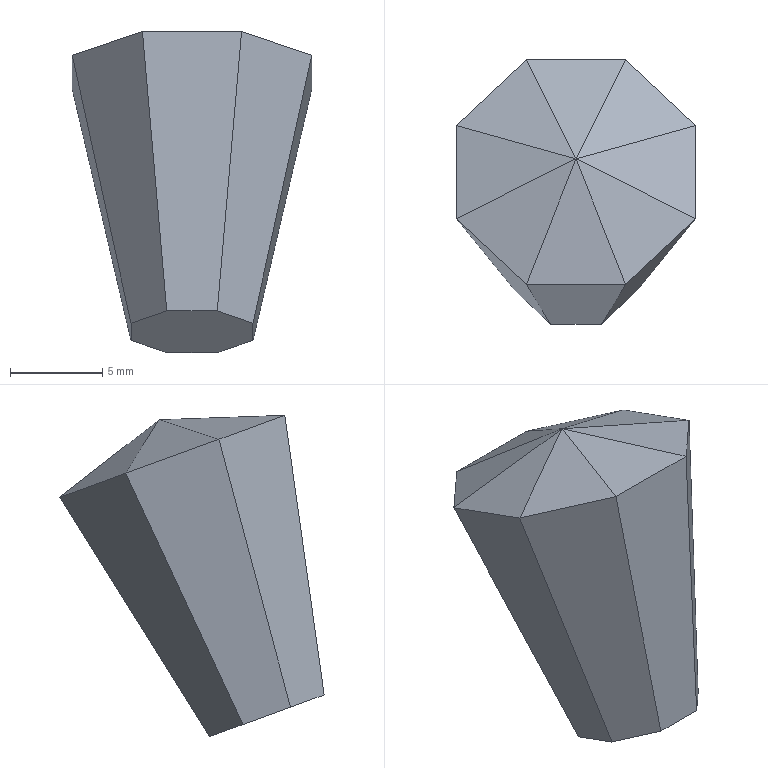Component | NX | MODEL27 | 1 solid | 17 faces | box 13 x 14.35 x 17.45 mm | volume 1338 mm3 | plane 17
STEP:
#1=CARTESIAN_POINT('',(0.,0.,0.));
#2=DIRECTION('',(0.,0.,1.));
#3=DIRECTION('',(1.,0.,0.));
#4=AXIS2_PLACEMENT_3D('',#1,#2,#3);
#5=CARTESIAN_POINT('',(-3.313,7.557,72.335));
#6=VERTEX_POINT('',#5);
#7=CARTESIAN_POINT('',(-3.313,4.978,73.273));
#8=VERTEX_POINT('',#7);
#9=CARTESIAN_POINT('',(-3.313,7.557,72.335));
#10=DIRECTION('',(-0.,-0.9397,0.342));
#11=VECTOR('',#10,1.);
#12=LINE('',#9,#11);
#13=CARTESIAN_POINT('',(-3.313,7.557,72.335));
#14=DIRECTION('',(0.9781,0.07111,0.1954));
#15=DIRECTION('',(0.2079,-0.3345,-0.9192));
#16=AXIS2_PLACEMENT_3D('',#13,#14,#15);
#17=PLANE('',#16);
#18=CARTESIAN_POINT('',(0.,0.));
#19=DIRECTION('',(0.,-1.));
#20=VECTOR('',#19,1.);
#21=LINE('',#18,#20);
#22=(GEOMETRIC_REPRESENTATION_CONTEXT(2)PARAMETRIC_REPRESENTATION_CONTEXT()REPRESENTATION_CONTEXT('',''));
#23=DEFINITIONAL_REPRESENTATION('',(#21),#22);
#24=PCURVE('',#17,#23);
#25=CARTESIAN_POINT('',(0.,6.268,72.804));
#26=DIRECTION('',(0.,0.342,0.9397));
#27=DIRECTION('',(1.,0.,0.));
#28=AXIS2_PLACEMENT_3D('',#25,#26,#27);
#29=PLANE('',#28);
#30=CARTESIAN_POINT('',(-3.313,1.372));
#31=DIRECTION('',(-0.,-1.));
#32=VECTOR('',#31,1.);
#33=LINE('',#30,#32);
#34=(GEOMETRIC_REPRESENTATION_CONTEXT(2)PARAMETRIC_REPRESENTATION_CONTEXT()REPRESENTATION_CONTEXT('',''));
#35=DEFINITIONAL_REPRESENTATION('',(#33),#34);
#36=PCURVE('',#29,#35);
#37=SURFACE_CURVE('',#12,(#24,#36),.PCURVE_S1.);
#38=EDGE_CURVE('',#6,#8,#37,.T.);
#39=ORIENTED_EDGE('',*,*,#38,.T.);
#40=CARTESIAN_POINT('',(-6.502,8.867,87.821));
#41=VERTEX_POINT('',#40);
#42=CARTESIAN_POINT('',(-3.313,4.978,73.273));
#43=DIRECTION('',(0.2071,-0.2527,-0.9451));
#44=VECTOR('',#43,1.);
#45=LINE('',#42,#44);
#46=CARTESIAN_POINT('',(0.,-2.745));
#47=DIRECTION('',(0.9963,0.0858));
#48=VECTOR('',#47,1.);
#49=LINE('',#46,#48);
#50=(GEOMETRIC_REPRESENTATION_CONTEXT(2)PARAMETRIC_REPRESENTATION_CONTEXT()REPRESENTATION_CONTEXT('',''));
#51=DEFINITIONAL_REPRESENTATION('',(#49),#50);
#52=PCURVE('',#17,#51);
#53=CARTESIAN_POINT('',(-3.313,4.978,73.273));
#54=DIRECTION('',(0.6917,0.7211,-0.04119));
#55=DIRECTION('',(-0.7071,0.6645,-0.2418));
#56=AXIS2_PLACEMENT_3D('',#53,#54,#55);
#57=PLANE('',#56);
#58=CARTESIAN_POINT('',(0.,0.));
#59=DIRECTION('',(-0.0858,-0.9963));
#60=VECTOR('',#59,1.);
#61=LINE('',#58,#60);
#62=(GEOMETRIC_REPRESENTATION_CONTEXT(2)PARAMETRIC_REPRESENTATION_CONTEXT()REPRESENTATION_CONTEXT('',''));
#63=DEFINITIONAL_REPRESENTATION('',(#61),#62);
#64=PCURVE('',#57,#63);
#65=SURFACE_CURVE('',#45,(#52,#64),.PCURVE_S1.);
#66=EDGE_CURVE('',#41,#8,#65,.T.);
#67=ORIENTED_EDGE('',*,*,#66,.F.);
#68=CARTESIAN_POINT('',(-6.502,13.929,85.978));
#69=VERTEX_POINT('',#68);
#70=CARTESIAN_POINT('',(-6.502,12.688,86.43));
#71=DIRECTION('',(-0.,-0.9397,0.342));
#72=VECTOR('',#71,1.);
#73=LINE('',#70,#72);
#74=CARTESIAN_POINT('',(-15.335,-0.));
#75=DIRECTION('',(0.,-1.));
#76=VECTOR('',#75,1.);
#77=LINE('',#74,#76);
#78=(GEOMETRIC_REPRESENTATION_CONTEXT(2)PARAMETRIC_REPRESENTATION_CONTEXT()REPRESENTATION_CONTEXT('',''));
#79=DEFINITIONAL_REPRESENTATION('',(#77),#78);
#80=PCURVE('',#17,#79);
#81=CARTESIAN_POINT('',(-6.502,13.929,85.978));
#82=DIRECTION('',(-0.309,0.3253,0.8937));
#83=DIRECTION('',(0.9511,0.1057,0.2904));
#84=AXIS2_PLACEMENT_3D('',#81,#82,#83);
#85=PLANE('',#84);
#86=CARTESIAN_POINT('',(-0.,-1.321));
#87=DIRECTION('',(-0.,-1.));
#88=VECTOR('',#87,1.);
#89=LINE('',#86,#88);
#90=(GEOMETRIC_REPRESENTATION_CONTEXT(2)PARAMETRIC_REPRESENTATION_CONTEXT()REPRESENTATION_CONTEXT('',''));
#91=DEFINITIONAL_REPRESENTATION('',(#89),#90);
#92=PCURVE('',#85,#91);
#93=SURFACE_CURVE('',#73,(#80,#92),.PCURVE_S1.);
#94=EDGE_CURVE('',#69,#41,#93,.T.);
#95=ORIENTED_EDGE('',*,*,#94,.F.);
#96=CARTESIAN_POINT('',(-3.313,7.557,72.335));
#97=DIRECTION('',(0.2071,-0.4139,-0.8864));
#98=VECTOR('',#97,1.);
#99=LINE('',#96,#98);
#100=CARTESIAN_POINT('',(0.,0.));
#101=DIRECTION('',(0.9963,-0.0858));
#102=VECTOR('',#101,1.);
#103=LINE('',#100,#102);
#104=(GEOMETRIC_REPRESENTATION_CONTEXT(2)PARAMETRIC_REPRESENTATION_CONTEXT()REPRESENTATION_CONTEXT('',''));
#105=DEFINITIONAL_REPRESENTATION('',(#103),#104);
#106=PCURVE('',#17,#105);
#107=CARTESIAN_POINT('',(-1.372,9.381,71.671));
#108=DIRECTION('',(0.6917,-0.5788,0.4319));
#109=DIRECTION('',(0.7071,0.6645,-0.2418));
#110=AXIS2_PLACEMENT_3D('',#107,#108,#109);
#111=PLANE('',#110);
#112=CARTESIAN_POINT('',(-2.745,0.));
#113=DIRECTION('',(0.0858,-0.9963));
#114=VECTOR('',#113,1.);
#115=LINE('',#112,#114);
#116=(GEOMETRIC_REPRESENTATION_CONTEXT(2)PARAMETRIC_REPRESENTATION_CONTEXT()REPRESENTATION_CONTEXT('',''));
#117=DEFINITIONAL_REPRESENTATION('',(#115),#116);
#118=PCURVE('',#111,#117);
#119=SURFACE_CURVE('',#99,(#106,#118),.PCURVE_S1.);
#120=EDGE_CURVE('',#69,#6,#119,.T.);
#121=ORIENTED_EDGE('',*,*,#120,.T.);
#122=EDGE_LOOP('',(#39,#67,#95,#121));
#123=FACE_BOUND('',#122,.T.);
#124=ADVANCED_FACE('',(#123),#17,.F.);
#125=CARTESIAN_POINT('',(-1.372,3.154,73.937));
#126=VERTEX_POINT('',#125);
#127=CARTESIAN_POINT('',(-3.313,4.978,73.273));
#128=DIRECTION('',(0.7071,-0.6645,0.2418));
#129=VECTOR('',#128,1.);
#130=LINE('',#127,#129);
#131=CARTESIAN_POINT('',(0.,0.));
#132=DIRECTION('',(-1.,-0.));
#133=VECTOR('',#132,1.);
#134=LINE('',#131,#133);
#135=(GEOMETRIC_REPRESENTATION_CONTEXT(2)PARAMETRIC_REPRESENTATION_CONTEXT()REPRESENTATION_CONTEXT('',''));
#136=DEFINITIONAL_REPRESENTATION('',(#134),#135);
#137=PCURVE('',#57,#136);
#138=CARTESIAN_POINT('',(-3.313,-1.372));
#139=DIRECTION('',(0.7071,-0.7071));
#140=VECTOR('',#139,1.);
#141=LINE('',#138,#140);
#142=(GEOMETRIC_REPRESENTATION_CONTEXT(2)PARAMETRIC_REPRESENTATION_CONTEXT()REPRESENTATION_CONTEXT('',''));
#143=DEFINITIONAL_REPRESENTATION('',(#141),#142);
#144=PCURVE('',#29,#143);
#145=SURFACE_CURVE('',#130,(#137,#144),.PCURVE_S1.);
#146=EDGE_CURVE('',#8,#126,#145,.T.);
#147=ORIENTED_EDGE('',*,*,#146,.T.);
#148=CARTESIAN_POINT('',(-2.693,5.288,89.123));
#149=VERTEX_POINT('',#148);
#150=CARTESIAN_POINT('',(-1.372,3.154,73.937));
#151=DIRECTION('',(0.0858,-0.1387,-0.9866));
#152=VECTOR('',#151,1.);
#153=LINE('',#150,#152);
#154=CARTESIAN_POINT('',(-2.745,0.));
#155=DIRECTION('',(0.0858,-0.9963));
#156=VECTOR('',#155,1.);
#157=LINE('',#154,#156);
#158=(GEOMETRIC_REPRESENTATION_CONTEXT(2)PARAMETRIC_REPRESENTATION_CONTEXT()REPRESENTATION_CONTEXT('',''));
#159=DEFINITIONAL_REPRESENTATION('',(#157),#158);
#160=PCURVE('',#57,#159);
#161=CARTESIAN_POINT('',(-1.372,3.154,73.937));
#162=DIRECTION('',(0.,0.9903,-0.1392));
#163=DIRECTION('',(0.,0.1392,0.9903));
#164=AXIS2_PLACEMENT_3D('',#161,#162,#163);
#165=PLANE('',#164);
#166=CARTESIAN_POINT('',(0.,0.));
#167=DIRECTION('',(-0.9963,0.0858));
#168=VECTOR('',#167,1.);
#169=LINE('',#166,#168);
#170=(GEOMETRIC_REPRESENTATION_CONTEXT(2)PARAMETRIC_REPRESENTATION_CONTEXT()REPRESENTATION_CONTEXT('',''));
#171=DEFINITIONAL_REPRESENTATION('',(#169),#170);
#172=PCURVE('',#165,#171);
#173=SURFACE_CURVE('',#153,(#160,#172),.PCURVE_S1.);
#174=EDGE_CURVE('',#149,#126,#173,.T.);
#175=ORIENTED_EDGE('',*,*,#174,.F.);
#176=CARTESIAN_POINT('',(-5.568,7.99,88.14));
#177=DIRECTION('',(0.7071,-0.6645,0.2418));
#178=VECTOR('',#177,1.);
#179=LINE('',#176,#178);
#180=CARTESIAN_POINT('',(-0.,15.335));
#181=DIRECTION('',(-1.,-0.));
#182=VECTOR('',#181,1.);
#183=LINE('',#180,#182);
#184=(GEOMETRIC_REPRESENTATION_CONTEXT(2)PARAMETRIC_REPRESENTATION_CONTEXT()REPRESENTATION_CONTEXT('',''));
#185=DEFINITIONAL_REPRESENTATION('',(#183),#184);
#186=PCURVE('',#57,#185);
#187=CARTESIAN_POINT('',(-6.502,8.867,87.821));
#188=DIRECTION('',(-0.2185,0.12,0.9684));
#189=DIRECTION('',(0.9746,0.07658,0.2104));
#190=AXIS2_PLACEMENT_3D('',#187,#188,#189);
#191=PLANE('',#190);
#192=CARTESIAN_POINT('',(0.9101,-0.957));
#193=DIRECTION('',(0.6892,-0.7246));
#194=VECTOR('',#193,1.);
#195=LINE('',#192,#194);
#196=(GEOMETRIC_REPRESENTATION_CONTEXT(2)PARAMETRIC_REPRESENTATION_CONTEXT()REPRESENTATION_CONTEXT('',''));
#197=DEFINITIONAL_REPRESENTATION('',(#195),#196);
#198=PCURVE('',#191,#197);
#199=SURFACE_CURVE('',#179,(#186,#198),.PCURVE_S1.);
#200=EDGE_CURVE('',#41,#149,#199,.T.);
#201=ORIENTED_EDGE('',*,*,#200,.F.);
#202=ORIENTED_EDGE('',*,*,#66,.T.);
#203=EDGE_LOOP('',(#147,#175,#201,#202));
#204=FACE_BOUND('',#203,.T.);
#205=ADVANCED_FACE('',(#204),#57,.F.);
#206=CARTESIAN_POINT('',(1.372,3.154,73.937));
#207=VERTEX_POINT('',#206);
#208=CARTESIAN_POINT('',(-1.372,3.154,73.937));
#209=DIRECTION('',(1.,0.,0.));
#210=VECTOR('',#209,1.);
#211=LINE('',#208,#210);
#212=CARTESIAN_POINT('',(0.,0.));
#213=DIRECTION('',(0.,1.));
#214=VECTOR('',#213,1.);
#215=LINE('',#212,#214);
#216=(GEOMETRIC_REPRESENTATION_CONTEXT(2)PARAMETRIC_REPRESENTATION_CONTEXT()REPRESENTATION_CONTEXT('',''));
#217=DEFINITIONAL_REPRESENTATION('',(#215),#216);
#218=PCURVE('',#165,#217);
#219=CARTESIAN_POINT('',(-1.372,-3.313));
#220=DIRECTION('',(1.,0.));
#221=VECTOR('',#220,1.);
#222=LINE('',#219,#221);
#223=(GEOMETRIC_REPRESENTATION_CONTEXT(2)PARAMETRIC_REPRESENTATION_CONTEXT()REPRESENTATION_CONTEXT('',''));
#224=DEFINITIONAL_REPRESENTATION('',(#222),#223);
#225=PCURVE('',#29,#224);
#226=SURFACE_CURVE('',#211,(#218,#225),.PCURVE_S1.);
#227=EDGE_CURVE('',#126,#207,#226,.T.);
#228=ORIENTED_EDGE('',*,*,#227,.T.);
#229=CARTESIAN_POINT('',(2.693,5.288,89.123));
#230=VERTEX_POINT('',#229);
#231=CARTESIAN_POINT('',(1.372,3.154,73.937));
#232=DIRECTION('',(-0.0858,-0.1387,-0.9866));
#233=VECTOR('',#232,1.);
#234=LINE('',#231,#233);
#235=CARTESIAN_POINT('',(0.,2.745));
#236=DIRECTION('',(-0.9963,-0.0858));
#237=VECTOR('',#236,1.);
#238=LINE('',#235,#237);
#239=(GEOMETRIC_REPRESENTATION_CONTEXT(2)PARAMETRIC_REPRESENTATION_CONTEXT()REPRESENTATION_CONTEXT('',''));
#240=DEFINITIONAL_REPRESENTATION('',(#238),#239);
#241=PCURVE('',#165,#240);
#242=CARTESIAN_POINT('',(1.372,3.154,73.937));
#243=DIRECTION('',(-0.6917,0.7211,-0.04119));
#244=DIRECTION('',(-0.7071,-0.6645,0.2418));
#245=AXIS2_PLACEMENT_3D('',#242,#243,#244);
#246=PLANE('',#245);
#247=CARTESIAN_POINT('',(0.,0.));
#248=DIRECTION('',(-0.0858,-0.9963));
#249=VECTOR('',#248,1.);
#250=LINE('',#247,#249);
#251=(GEOMETRIC_REPRESENTATION_CONTEXT(2)PARAMETRIC_REPRESENTATION_CONTEXT()REPRESENTATION_CONTEXT('',''));
#252=DEFINITIONAL_REPRESENTATION('',(#250),#251);
#253=PCURVE('',#246,#252);
#254=SURFACE_CURVE('',#234,(#241,#253),.PCURVE_S1.);
#255=EDGE_CURVE('',#230,#207,#254,.T.);
#256=ORIENTED_EDGE('',*,*,#255,.F.);
#257=CARTESIAN_POINT('',(-1.372,5.288,89.123));
#258=DIRECTION('',(1.,0.,0.));
#259=VECTOR('',#258,1.);
#260=LINE('',#257,#259);
#261=CARTESIAN_POINT('',(15.335,0.));
#262=DIRECTION('',(0.,1.));
#263=VECTOR('',#262,1.);
#264=LINE('',#261,#263);
#265=(GEOMETRIC_REPRESENTATION_CONTEXT(2)PARAMETRIC_REPRESENTATION_CONTEXT()REPRESENTATION_CONTEXT('',''));
#266=DEFINITIONAL_REPRESENTATION('',(#264),#265);
#267=PCURVE('',#165,#266);
#268=CARTESIAN_POINT('',(-2.693,5.288,89.123));
#269=DIRECTION('',(0.,0.0349,0.9994));
#270=DIRECTION('',(0.,-0.9994,0.0349));
#271=AXIS2_PLACEMENT_3D('',#268,#269,#270);
#272=PLANE('',#271);
#273=CARTESIAN_POINT('',(0.,1.321));
#274=DIRECTION('',(0.,1.));
#275=VECTOR('',#274,1.);
#276=LINE('',#273,#275);
#277=(GEOMETRIC_REPRESENTATION_CONTEXT(2)PARAMETRIC_REPRESENTATION_CONTEXT()REPRESENTATION_CONTEXT('',''));
#278=DEFINITIONAL_REPRESENTATION('',(#276),#277);
#279=PCURVE('',#272,#278);
#280=SURFACE_CURVE('',#260,(#267,#279),.PCURVE_S1.);
#281=EDGE_CURVE('',#149,#230,#280,.T.);
#282=ORIENTED_EDGE('',*,*,#281,.F.);
#283=ORIENTED_EDGE('',*,*,#174,.T.);
#284=EDGE_LOOP('',(#228,#256,#282,#283));
#285=FACE_BOUND('',#284,.T.);
#286=ADVANCED_FACE('',(#285),#165,.F.);
#287=CARTESIAN_POINT('',(3.313,4.978,73.273));
#288=VERTEX_POINT('',#287);
#289=CARTESIAN_POINT('',(1.372,3.154,73.937));
#290=DIRECTION('',(0.7071,0.6645,-0.2418));
#291=VECTOR('',#290,1.);
#292=LINE('',#289,#291);
#293=CARTESIAN_POINT('',(0.,0.));
#294=DIRECTION('',(-1.,0.));
#295=VECTOR('',#294,1.);
#296=LINE('',#293,#295);
#297=(GEOMETRIC_REPRESENTATION_CONTEXT(2)PARAMETRIC_REPRESENTATION_CONTEXT()REPRESENTATION_CONTEXT('',''));
#298=DEFINITIONAL_REPRESENTATION('',(#296),#297);
#299=PCURVE('',#246,#298);
#300=CARTESIAN_POINT('',(1.372,-3.313));
#301=DIRECTION('',(0.7071,0.7071));
#302=VECTOR('',#301,1.);
#303=LINE('',#300,#302);
#304=(GEOMETRIC_REPRESENTATION_CONTEXT(2)PARAMETRIC_REPRESENTATION_CONTEXT()REPRESENTATION_CONTEXT('',''));
#305=DEFINITIONAL_REPRESENTATION('',(#303),#304);
#306=PCURVE('',#29,#305);
#307=SURFACE_CURVE('',#292,(#299,#306),.PCURVE_S1.);
#308=EDGE_CURVE('',#207,#288,#307,.T.);
#309=ORIENTED_EDGE('',*,*,#308,.T.);
#310=CARTESIAN_POINT('',(6.502,8.867,87.821));
#311=VERTEX_POINT('',#310);
#312=CARTESIAN_POINT('',(3.313,4.978,73.273));
#313=DIRECTION('',(-0.2071,-0.2527,-0.9451));
#314=VECTOR('',#313,1.);
#315=LINE('',#312,#314);
#316=CARTESIAN_POINT('',(-2.745,-0.));
#317=DIRECTION('',(0.0858,-0.9963));
#318=VECTOR('',#317,1.);
#319=LINE('',#316,#318);
#320=(GEOMETRIC_REPRESENTATION_CONTEXT(2)PARAMETRIC_REPRESENTATION_CONTEXT()REPRESENTATION_CONTEXT('',''));
#321=DEFINITIONAL_REPRESENTATION('',(#319),#320);
#322=PCURVE('',#246,#321);
#323=CARTESIAN_POINT('',(3.313,4.978,73.273));
#324=DIRECTION('',(-0.9781,0.07111,0.1954));
#325=DIRECTION('',(0.2079,0.3345,0.9192));
#326=AXIS2_PLACEMENT_3D('',#323,#324,#325);
#327=PLANE('',#326);
#328=CARTESIAN_POINT('',(0.,0.));
#329=DIRECTION('',(-0.9963,0.0858));
#330=VECTOR('',#329,1.);
#331=LINE('',#328,#330);
#332=(GEOMETRIC_REPRESENTATION_CONTEXT(2)PARAMETRIC_REPRESENTATION_CONTEXT()REPRESENTATION_CONTEXT('',''));
#333=DEFINITIONAL_REPRESENTATION('',(#331),#332);
#334=PCURVE('',#327,#333);
#335=SURFACE_CURVE('',#315,(#322,#334),.PCURVE_S1.);
#336=EDGE_CURVE('',#311,#288,#335,.T.);
#337=ORIENTED_EDGE('',*,*,#336,.F.);
#338=CARTESIAN_POINT('',(3.627,6.166,88.804));
#339=DIRECTION('',(0.7071,0.6645,-0.2418));
#340=VECTOR('',#339,1.);
#341=LINE('',#338,#340);
#342=CARTESIAN_POINT('',(0.,15.335));
#343=DIRECTION('',(-1.,0.));
#344=VECTOR('',#343,1.);
#345=LINE('',#342,#344);
#346=(GEOMETRIC_REPRESENTATION_CONTEXT(2)PARAMETRIC_REPRESENTATION_CONTEXT()REPRESENTATION_CONTEXT('',''));
#347=DEFINITIONAL_REPRESENTATION('',(#345),#346);
#348=PCURVE('',#246,#347);
#349=CARTESIAN_POINT('',(2.693,5.288,89.123));
#350=DIRECTION('',(0.2185,0.12,0.9684));
#351=DIRECTION('',(0.,-0.9924,0.1229));
#352=AXIS2_PLACEMENT_3D('',#349,#350,#351);
#353=PLANE('',#352);
#354=CARTESIAN_POINT('',(-0.9101,0.957));
#355=DIRECTION('',(-0.6892,0.7246));
#356=VECTOR('',#355,1.);
#357=LINE('',#354,#356);
#358=(GEOMETRIC_REPRESENTATION_CONTEXT(2)PARAMETRIC_REPRESENTATION_CONTEXT()REPRESENTATION_CONTEXT('',''));
#359=DEFINITIONAL_REPRESENTATION('',(#357),#358);
#360=PCURVE('',#353,#359);
#361=SURFACE_CURVE('',#341,(#348,#360),.PCURVE_S1.);
#362=EDGE_CURVE('',#230,#311,#361,.T.);
#363=ORIENTED_EDGE('',*,*,#362,.F.);
#364=ORIENTED_EDGE('',*,*,#255,.T.);
#365=EDGE_LOOP('',(#309,#337,#363,#364));
#366=FACE_BOUND('',#365,.T.);
#367=ADVANCED_FACE('',(#366),#246,.F.);
#368=CARTESIAN_POINT('',(3.313,7.557,72.335));
#369=VERTEX_POINT('',#368);
#370=CARTESIAN_POINT('',(3.313,4.978,73.273));
#371=DIRECTION('',(0.,0.9397,-0.342));
#372=VECTOR('',#371,1.);
#373=LINE('',#370,#372);
#374=CARTESIAN_POINT('',(0.,0.));
#375=DIRECTION('',(0.,1.));
#376=VECTOR('',#375,1.);
#377=LINE('',#374,#376);
#378=(GEOMETRIC_REPRESENTATION_CONTEXT(2)PARAMETRIC_REPRESENTATION_CONTEXT()REPRESENTATION_CONTEXT('',''));
#379=DEFINITIONAL_REPRESENTATION('',(#377),#378);
#380=PCURVE('',#327,#379);
#381=CARTESIAN_POINT('',(3.313,-1.372));
#382=DIRECTION('',(0.,1.));
#383=VECTOR('',#382,1.);
#384=LINE('',#381,#383);
#385=(GEOMETRIC_REPRESENTATION_CONTEXT(2)PARAMETRIC_REPRESENTATION_CONTEXT()REPRESENTATION_CONTEXT('',''));
#386=DEFINITIONAL_REPRESENTATION('',(#384),#385);
#387=PCURVE('',#29,#386);
#388=SURFACE_CURVE('',#373,(#380,#387),.PCURVE_S1.);
#389=EDGE_CURVE('',#288,#369,#388,.T.);
#390=ORIENTED_EDGE('',*,*,#389,.T.);
#391=CARTESIAN_POINT('',(6.502,13.929,85.978));
#392=VERTEX_POINT('',#391);
#393=CARTESIAN_POINT('',(3.313,7.557,72.335));
#394=DIRECTION('',(-0.2071,-0.4139,-0.8864));
#395=VECTOR('',#394,1.);
#396=LINE('',#393,#395);
#397=CARTESIAN_POINT('',(0.,2.745));
#398=DIRECTION('',(-0.9963,-0.0858));
#399=VECTOR('',#398,1.);
#400=LINE('',#397,#399);
#401=(GEOMETRIC_REPRESENTATION_CONTEXT(2)PARAMETRIC_REPRESENTATION_CONTEXT()REPRESENTATION_CONTEXT('',''));
#402=DEFINITIONAL_REPRESENTATION('',(#400),#401);
#403=PCURVE('',#327,#402);
#404=CARTESIAN_POINT('',(3.313,7.557,72.335));
#405=DIRECTION('',(-0.6917,-0.5788,0.4319));
#406=DIRECTION('',(0.7071,-0.6645,0.2418));
#407=AXIS2_PLACEMENT_3D('',#404,#405,#406);
#408=PLANE('',#407);
#409=CARTESIAN_POINT('',(0.,0.));
#410=DIRECTION('',(-0.0858,-0.9963));
#411=VECTOR('',#410,1.);
#412=LINE('',#409,#411);
#413=(GEOMETRIC_REPRESENTATION_CONTEXT(2)PARAMETRIC_REPRESENTATION_CONTEXT()REPRESENTATION_CONTEXT('',''));
#414=DEFINITIONAL_REPRESENTATION('',(#412),#413);
#415=PCURVE('',#408,#414);
#416=SURFACE_CURVE('',#396,(#403,#415),.PCURVE_S1.);
#417=EDGE_CURVE('',#392,#369,#416,.T.);
#418=ORIENTED_EDGE('',*,*,#417,.F.);
#419=CARTESIAN_POINT('',(6.502,10.108,87.369));
#420=DIRECTION('',(0.,0.9397,-0.342));
#421=VECTOR('',#420,1.);
#422=LINE('',#419,#421);
#423=CARTESIAN_POINT('',(15.335,-0.));
#424=DIRECTION('',(0.,1.));
#425=VECTOR('',#424,1.);
#426=LINE('',#423,#425);
#427=(GEOMETRIC_REPRESENTATION_CONTEXT(2)PARAMETRIC_REPRESENTATION_CONTEXT()REPRESENTATION_CONTEXT('',''));
#428=DEFINITIONAL_REPRESENTATION('',(#426),#427);
#429=PCURVE('',#327,#428);
#430=CARTESIAN_POINT('',(6.502,8.867,87.821));
#431=DIRECTION('',(0.309,0.3253,0.8937));
#432=DIRECTION('',(0.9511,-0.1057,-0.2904));
#433=AXIS2_PLACEMENT_3D('',#430,#431,#432);
#434=PLANE('',#433);
#435=CARTESIAN_POINT('',(0.,1.321));
#436=DIRECTION('',(0.,1.));
#437=VECTOR('',#436,1.);
#438=LINE('',#435,#437);
#439=(GEOMETRIC_REPRESENTATION_CONTEXT(2)PARAMETRIC_REPRESENTATION_CONTEXT()REPRESENTATION_CONTEXT('',''));
#440=DEFINITIONAL_REPRESENTATION('',(#438),#439);
#441=PCURVE('',#434,#440);
#442=SURFACE_CURVE('',#422,(#429,#441),.PCURVE_S1.);
#443=EDGE_CURVE('',#311,#392,#442,.T.);
#444=ORIENTED_EDGE('',*,*,#443,.F.);
#445=ORIENTED_EDGE('',*,*,#336,.T.);
#446=EDGE_LOOP('',(#390,#418,#444,#445));
#447=FACE_BOUND('',#446,.T.);
#448=ADVANCED_FACE('',(#447),#327,.F.);
#449=CARTESIAN_POINT('',(1.372,9.381,71.671));
#450=VERTEX_POINT('',#449);
#451=CARTESIAN_POINT('',(3.313,7.557,72.335));
#452=DIRECTION('',(-0.7071,0.6645,-0.2418));
#453=VECTOR('',#452,1.);
#454=LINE('',#451,#453);
#455=CARTESIAN_POINT('',(0.,0.));
#456=DIRECTION('',(-1.,0.));
#457=VECTOR('',#456,1.);
#458=LINE('',#455,#457);
#459=(GEOMETRIC_REPRESENTATION_CONTEXT(2)PARAMETRIC_REPRESENTATION_CONTEXT()REPRESENTATION_CONTEXT('',''));
#460=DEFINITIONAL_REPRESENTATION('',(#458),#459);
#461=PCURVE('',#408,#460);
#462=CARTESIAN_POINT('',(3.313,1.372));
#463=DIRECTION('',(-0.7071,0.7071));
#464=VECTOR('',#463,1.);
#465=LINE('',#462,#464);
#466=(GEOMETRIC_REPRESENTATION_CONTEXT(2)PARAMETRIC_REPRESENTATION_CONTEXT()REPRESENTATION_CONTEXT('',''));
#467=DEFINITIONAL_REPRESENTATION('',(#465),#466);
#468=PCURVE('',#29,#467);
#469=SURFACE_CURVE('',#454,(#461,#468),.PCURVE_S1.);
#470=EDGE_CURVE('',#369,#450,#469,.T.);
#471=ORIENTED_EDGE('',*,*,#470,.T.);
#472=CARTESIAN_POINT('',(2.693,17.508,84.676));
#473=VERTEX_POINT('',#472);
#474=CARTESIAN_POINT('',(1.372,9.381,71.671));
#475=DIRECTION('',(-0.0858,-0.528,-0.8449));
#476=VECTOR('',#475,1.);
#477=LINE('',#474,#476);
#478=CARTESIAN_POINT('',(-2.745,-0.));
#479=DIRECTION('',(0.0858,-0.9963));
#480=VECTOR('',#479,1.);
#481=LINE('',#478,#480);
#482=(GEOMETRIC_REPRESENTATION_CONTEXT(2)PARAMETRIC_REPRESENTATION_CONTEXT()REPRESENTATION_CONTEXT('',''));
#483=DEFINITIONAL_REPRESENTATION('',(#481),#482);
#484=PCURVE('',#408,#483);
#485=CARTESIAN_POINT('',(1.372,9.381,71.671));
#486=DIRECTION('',(-0.,-0.848,0.5299));
#487=DIRECTION('',(0.,-0.5299,-0.848));
#488=AXIS2_PLACEMENT_3D('',#485,#486,#487);
#489=PLANE('',#488);
#490=CARTESIAN_POINT('',(0.,0.));
#491=DIRECTION('',(0.9963,-0.0858));
#492=VECTOR('',#491,1.);
#493=LINE('',#490,#492);
#494=(GEOMETRIC_REPRESENTATION_CONTEXT(2)PARAMETRIC_REPRESENTATION_CONTEXT()REPRESENTATION_CONTEXT('',''));
#495=DEFINITIONAL_REPRESENTATION('',(#493),#494);
#496=PCURVE('',#489,#495);
#497=SURFACE_CURVE('',#477,(#484,#496),.PCURVE_S1.);
#498=EDGE_CURVE('',#473,#450,#497,.T.);
#499=ORIENTED_EDGE('',*,*,#498,.F.);
#500=CARTESIAN_POINT('',(5.568,14.806,85.659));
#501=DIRECTION('',(-0.7071,0.6645,-0.2418));
#502=VECTOR('',#501,1.);
#503=LINE('',#500,#502);
#504=CARTESIAN_POINT('',(0.,15.335));
#505=DIRECTION('',(-1.,0.));
#506=VECTOR('',#505,1.);
#507=LINE('',#504,#506);
#508=(GEOMETRIC_REPRESENTATION_CONTEXT(2)PARAMETRIC_REPRESENTATION_CONTEXT()REPRESENTATION_CONTEXT('',''));
#509=DEFINITIONAL_REPRESENTATION('',(#507),#508);
#510=PCURVE('',#408,#509);
#511=CARTESIAN_POINT('',(6.502,13.929,85.978));
#512=DIRECTION('',(0.2185,0.5306,0.819));
#513=DIRECTION('',(0.9746,-0.07658,-0.2104));
#514=AXIS2_PLACEMENT_3D('',#511,#512,#513);
#515=PLANE('',#514);
#516=CARTESIAN_POINT('',(-0.9101,0.957));
#517=DIRECTION('',(-0.6892,0.7246));
#518=VECTOR('',#517,1.);
#519=LINE('',#516,#518);
#520=(GEOMETRIC_REPRESENTATION_CONTEXT(2)PARAMETRIC_REPRESENTATION_CONTEXT()REPRESENTATION_CONTEXT('',''));
#521=DEFINITIONAL_REPRESENTATION('',(#519),#520);
#522=PCURVE('',#515,#521);
#523=SURFACE_CURVE('',#503,(#510,#522),.PCURVE_S1.);
#524=EDGE_CURVE('',#392,#473,#523,.T.);
#525=ORIENTED_EDGE('',*,*,#524,.F.);
#526=ORIENTED_EDGE('',*,*,#417,.T.);
#527=EDGE_LOOP('',(#471,#499,#525,#526));
#528=FACE_BOUND('',#527,.T.);
#529=ADVANCED_FACE('',(#528),#408,.F.);
#530=CARTESIAN_POINT('',(-1.372,9.381,71.671));
#531=VERTEX_POINT('',#530);
#532=CARTESIAN_POINT('',(1.372,9.381,71.671));
#533=DIRECTION('',(-1.,0.,-0.));
#534=VECTOR('',#533,1.);
#535=LINE('',#532,#534);
#536=CARTESIAN_POINT('',(0.,0.));
#537=DIRECTION('',(-0.,-1.));
#538=VECTOR('',#537,1.);
#539=LINE('',#536,#538);
#540=(GEOMETRIC_REPRESENTATION_CONTEXT(2)PARAMETRIC_REPRESENTATION_CONTEXT()REPRESENTATION_CONTEXT('',''));
#541=DEFINITIONAL_REPRESENTATION('',(#539),#540);
#542=PCURVE('',#489,#541);
#543=CARTESIAN_POINT('',(1.372,3.313));
#544=DIRECTION('',(-1.,0.));
#545=VECTOR('',#544,1.);
#546=LINE('',#543,#545);
#547=(GEOMETRIC_REPRESENTATION_CONTEXT(2)PARAMETRIC_REPRESENTATION_CONTEXT()REPRESENTATION_CONTEXT('',''));
#548=DEFINITIONAL_REPRESENTATION('',(#546),#547);
#549=PCURVE('',#29,#548);
#550=SURFACE_CURVE('',#535,(#542,#549),.PCURVE_S1.);
#551=EDGE_CURVE('',#450,#531,#550,.T.);
#552=ORIENTED_EDGE('',*,*,#551,.T.);
#553=CARTESIAN_POINT('',(-2.693,17.508,84.676));
#554=VERTEX_POINT('',#553);
#555=CARTESIAN_POINT('',(-1.372,9.381,71.671));
#556=DIRECTION('',(0.0858,-0.528,-0.8449));
#557=VECTOR('',#556,1.);
#558=LINE('',#555,#557);
#559=CARTESIAN_POINT('',(-0.,-2.745));
#560=DIRECTION('',(0.9963,0.0858));
#561=VECTOR('',#560,1.);
#562=LINE('',#559,#561);
#563=(GEOMETRIC_REPRESENTATION_CONTEXT(2)PARAMETRIC_REPRESENTATION_CONTEXT()REPRESENTATION_CONTEXT('',''));
#564=DEFINITIONAL_REPRESENTATION('',(#562),#563);
#565=PCURVE('',#489,#564);
#566=CARTESIAN_POINT('',(0.,0.));
#567=DIRECTION('',(-0.0858,-0.9963));
#568=VECTOR('',#567,1.);
#569=LINE('',#566,#568);
#570=(GEOMETRIC_REPRESENTATION_CONTEXT(2)PARAMETRIC_REPRESENTATION_CONTEXT()REPRESENTATION_CONTEXT('',''));
#571=DEFINITIONAL_REPRESENTATION('',(#569),#570);
#572=PCURVE('',#111,#571);
#573=SURFACE_CURVE('',#558,(#565,#572),.PCURVE_S1.);
#574=EDGE_CURVE('',#554,#531,#573,.T.);
#575=ORIENTED_EDGE('',*,*,#574,.F.);
#576=CARTESIAN_POINT('',(1.372,17.508,84.676));
#577=DIRECTION('',(-1.,0.,-0.));
#578=VECTOR('',#577,1.);
#579=LINE('',#576,#578);
#580=CARTESIAN_POINT('',(-15.335,-0.));
#581=DIRECTION('',(-0.,-1.));
#582=VECTOR('',#581,1.);
#583=LINE('',#580,#582);
#584=(GEOMETRIC_REPRESENTATION_CONTEXT(2)PARAMETRIC_REPRESENTATION_CONTEXT()REPRESENTATION_CONTEXT('',''));
#585=DEFINITIONAL_REPRESENTATION('',(#583),#584);
#586=PCURVE('',#489,#585);
#587=CARTESIAN_POINT('',(2.693,17.508,84.676));
#588=DIRECTION('',(0.,0.6157,0.788));
#589=DIRECTION('',(0.,-0.788,0.6157));
#590=AXIS2_PLACEMENT_3D('',#587,#588,#589);
#591=PLANE('',#590);
#592=CARTESIAN_POINT('',(0.,-1.321));
#593=DIRECTION('',(-0.,-1.));
#594=VECTOR('',#593,1.);
#595=LINE('',#592,#594);
#596=(GEOMETRIC_REPRESENTATION_CONTEXT(2)PARAMETRIC_REPRESENTATION_CONTEXT()REPRESENTATION_CONTEXT('',''));
#597=DEFINITIONAL_REPRESENTATION('',(#595),#596);
#598=PCURVE('',#591,#597);
#599=SURFACE_CURVE('',#579,(#586,#598),.PCURVE_S1.);
#600=EDGE_CURVE('',#473,#554,#599,.T.);
#601=ORIENTED_EDGE('',*,*,#600,.F.);
#602=ORIENTED_EDGE('',*,*,#498,.T.);
#603=EDGE_LOOP('',(#552,#575,#601,#602));
#604=FACE_BOUND('',#603,.T.);
#605=ADVANCED_FACE('',(#604),#489,.F.);
#606=CARTESIAN_POINT('',(-1.372,9.381,71.671));
#607=DIRECTION('',(-0.7071,-0.6645,0.2418));
#608=VECTOR('',#607,1.);
#609=LINE('',#606,#608);
#610=CARTESIAN_POINT('',(0.,0.));
#611=DIRECTION('',(-1.,-0.));
#612=VECTOR('',#611,1.);
#613=LINE('',#610,#612);
#614=(GEOMETRIC_REPRESENTATION_CONTEXT(2)PARAMETRIC_REPRESENTATION_CONTEXT()REPRESENTATION_CONTEXT('',''));
#615=DEFINITIONAL_REPRESENTATION('',(#613),#614);
#616=PCURVE('',#111,#615);
#617=CARTESIAN_POINT('',(-1.372,3.313));
#618=DIRECTION('',(-0.7071,-0.7071));
#619=VECTOR('',#618,1.);
#620=LINE('',#617,#619);
#621=(GEOMETRIC_REPRESENTATION_CONTEXT(2)PARAMETRIC_REPRESENTATION_CONTEXT()REPRESENTATION_CONTEXT('',''));
#622=DEFINITIONAL_REPRESENTATION('',(#620),#621);
#623=PCURVE('',#29,#622);
#624=SURFACE_CURVE('',#609,(#616,#623),.PCURVE_S1.);
#625=EDGE_CURVE('',#531,#6,#624,.T.);
#626=ORIENTED_EDGE('',*,*,#625,.T.);
#627=ORIENTED_EDGE('',*,*,#120,.F.);
#628=CARTESIAN_POINT('',(-3.627,16.63,84.995));
#629=DIRECTION('',(-0.7071,-0.6645,0.2418));
#630=VECTOR('',#629,1.);
#631=LINE('',#628,#630);
#632=CARTESIAN_POINT('',(-0.,15.335));
#633=DIRECTION('',(-1.,-0.));
#634=VECTOR('',#633,1.);
#635=LINE('',#632,#634);
#636=(GEOMETRIC_REPRESENTATION_CONTEXT(2)PARAMETRIC_REPRESENTATION_CONTEXT()REPRESENTATION_CONTEXT('',''));
#637=DEFINITIONAL_REPRESENTATION('',(#635),#636);
#638=PCURVE('',#111,#637);
#639=CARTESIAN_POINT('',(-2.693,17.508,84.676));
#640=DIRECTION('',(-0.2185,0.5306,0.819));
#641=DIRECTION('',(0.,-0.8392,0.5438));
#642=AXIS2_PLACEMENT_3D('',#639,#640,#641);
#643=PLANE('',#642);
#644=CARTESIAN_POINT('',(0.9101,-0.957));
#645=DIRECTION('',(0.6892,-0.7246));
#646=VECTOR('',#645,1.);
#647=LINE('',#644,#646);
#648=(GEOMETRIC_REPRESENTATION_CONTEXT(2)PARAMETRIC_REPRESENTATION_CONTEXT()REPRESENTATION_CONTEXT('',''));
#649=DEFINITIONAL_REPRESENTATION('',(#647),#648);
#650=PCURVE('',#643,#649);
#651=SURFACE_CURVE('',#631,(#638,#650),.PCURVE_S1.);
#652=EDGE_CURVE('',#554,#69,#651,.T.);
#653=ORIENTED_EDGE('',*,*,#652,.F.);
#654=ORIENTED_EDGE('',*,*,#574,.T.);
#655=EDGE_LOOP('',(#626,#627,#653,#654));
#656=FACE_BOUND('',#655,.T.);
#657=ADVANCED_FACE('',(#656),#111,.F.);
#658=ORIENTED_EDGE('',*,*,#38,.F.);
#659=ORIENTED_EDGE('',*,*,#625,.F.);
#660=ORIENTED_EDGE('',*,*,#551,.F.);
#661=ORIENTED_EDGE('',*,*,#470,.F.);
#662=ORIENTED_EDGE('',*,*,#389,.F.);
#663=ORIENTED_EDGE('',*,*,#308,.F.);
#664=ORIENTED_EDGE('',*,*,#227,.F.);
#665=ORIENTED_EDGE('',*,*,#146,.F.);
#666=EDGE_LOOP('',(#658,#659,#660,#661,#662,#663,#664,#665));
#667=FACE_BOUND('',#666,.T.);
#668=ADVANCED_FACE('',(#667),#29,.F.);
#669=ORIENTED_EDGE('',*,*,#94,.T.);
#670=CARTESIAN_POINT('',(0.,12.12,88.885));
#671=VERTEX_POINT('',#670);
#672=CARTESIAN_POINT('',(-6.502,8.867,87.821));
#673=DIRECTION('',(-0.8849,-0.4428,-0.1448));
#674=VECTOR('',#673,1.);
#675=LINE('',#672,#674);
#676=CARTESIAN_POINT('',(0.,-5.386));
#677=DIRECTION('',(-0.9304,-0.3665));
#678=VECTOR('',#677,1.);
#679=LINE('',#676,#678);
#680=(GEOMETRIC_REPRESENTATION_CONTEXT(2)PARAMETRIC_REPRESENTATION_CONTEXT()REPRESENTATION_CONTEXT('',''));
#681=DEFINITIONAL_REPRESENTATION('',(#679),#680);
#682=PCURVE('',#85,#681);
#683=CARTESIAN_POINT('',(0.,0.));
#684=DIRECTION('',(-0.9268,-0.3756));
#685=VECTOR('',#684,1.);
#686=LINE('',#683,#685);
#687=(GEOMETRIC_REPRESENTATION_CONTEXT(2)PARAMETRIC_REPRESENTATION_CONTEXT()REPRESENTATION_CONTEXT('',''));
#688=DEFINITIONAL_REPRESENTATION('',(#686),#687);
#689=PCURVE('',#191,#688);
#690=SURFACE_CURVE('',#675,(#682,#689),.PCURVE_S1.);
#691=EDGE_CURVE('',#671,#41,#690,.T.);
#692=ORIENTED_EDGE('',*,*,#691,.F.);
#693=CARTESIAN_POINT('',(-6.502,13.929,85.978));
#694=DIRECTION('',(-0.8849,0.2461,-0.3955));
#695=VECTOR('',#694,1.);
#696=LINE('',#693,#695);
#697=CARTESIAN_POINT('',(0.,0.));
#698=DIRECTION('',(-0.9304,0.3665));
#699=VECTOR('',#698,1.);
#700=LINE('',#697,#699);
#701=(GEOMETRIC_REPRESENTATION_CONTEXT(2)PARAMETRIC_REPRESENTATION_CONTEXT()REPRESENTATION_CONTEXT('',''));
#702=DEFINITIONAL_REPRESENTATION('',(#700),#701);
#703=PCURVE('',#85,#702);
#704=CARTESIAN_POINT('',(3.712,-3.903));
#705=DIRECTION('',(-0.4216,-0.9068));
#706=VECTOR('',#705,1.);
#707=LINE('',#704,#706);
#708=(GEOMETRIC_REPRESENTATION_CONTEXT(2)PARAMETRIC_REPRESENTATION_CONTEXT()REPRESENTATION_CONTEXT('',''));
#709=DEFINITIONAL_REPRESENTATION('',(#707),#708);
#710=PCURVE('',#643,#709);
#711=SURFACE_CURVE('',#696,(#703,#710),.PCURVE_S1.);
#712=EDGE_CURVE('',#671,#69,#711,.T.);
#713=ORIENTED_EDGE('',*,*,#712,.T.);
#714=EDGE_LOOP('',(#669,#692,#713));
#715=FACE_BOUND('',#714,.T.);
#716=ADVANCED_FACE('',(#715),#85,.T.);
#717=ORIENTED_EDGE('',*,*,#200,.T.);
#718=CARTESIAN_POINT('',(-2.693,5.288,89.123));
#719=DIRECTION('',(-0.3665,-0.9298,0.03247));
#720=VECTOR('',#719,1.);
#721=LINE('',#718,#720);
#722=CARTESIAN_POINT('',(3.712,-3.903));
#723=DIRECTION('',(-0.4216,-0.9068));
#724=VECTOR('',#723,1.);
#725=LINE('',#722,#724);
#726=(GEOMETRIC_REPRESENTATION_CONTEXT(2)PARAMETRIC_REPRESENTATION_CONTEXT()REPRESENTATION_CONTEXT('',''));
#727=DEFINITIONAL_REPRESENTATION('',(#725),#726);
#728=PCURVE('',#191,#727);
#729=CARTESIAN_POINT('',(0.,0.));
#730=DIRECTION('',(0.9304,-0.3665));
#731=VECTOR('',#730,1.);
#732=LINE('',#729,#731);
#733=(GEOMETRIC_REPRESENTATION_CONTEXT(2)PARAMETRIC_REPRESENTATION_CONTEXT()REPRESENTATION_CONTEXT('',''));
#734=DEFINITIONAL_REPRESENTATION('',(#732),#733);
#735=PCURVE('',#272,#734);
#736=SURFACE_CURVE('',#721,(#728,#735),.PCURVE_S1.);
#737=EDGE_CURVE('',#671,#149,#736,.T.);
#738=ORIENTED_EDGE('',*,*,#737,.F.);
#739=ORIENTED_EDGE('',*,*,#691,.T.);
#740=EDGE_LOOP('',(#717,#738,#739));
#741=FACE_BOUND('',#740,.T.);
#742=ADVANCED_FACE('',(#741),#191,.T.);
#743=ORIENTED_EDGE('',*,*,#281,.T.);
#744=CARTESIAN_POINT('',(2.693,5.288,89.123));
#745=DIRECTION('',(0.3665,-0.9298,0.03247));
#746=VECTOR('',#745,1.);
#747=LINE('',#744,#746);
#748=CARTESIAN_POINT('',(0.,5.386));
#749=DIRECTION('',(0.9304,0.3665));
#750=VECTOR('',#749,1.);
#751=LINE('',#748,#750);
#752=(GEOMETRIC_REPRESENTATION_CONTEXT(2)PARAMETRIC_REPRESENTATION_CONTEXT()REPRESENTATION_CONTEXT('',''));
#753=DEFINITIONAL_REPRESENTATION('',(#751),#752);
#754=PCURVE('',#272,#753);
#755=CARTESIAN_POINT('',(0.,0.));
#756=DIRECTION('',(0.9268,0.3756));
#757=VECTOR('',#756,1.);
#758=LINE('',#755,#757);
#759=(GEOMETRIC_REPRESENTATION_CONTEXT(2)PARAMETRIC_REPRESENTATION_CONTEXT()REPRESENTATION_CONTEXT('',''));
#760=DEFINITIONAL_REPRESENTATION('',(#758),#759);
#761=PCURVE('',#353,#760);
#762=SURFACE_CURVE('',#747,(#754,#761),.PCURVE_S1.);
#763=EDGE_CURVE('',#671,#230,#762,.T.);
#764=ORIENTED_EDGE('',*,*,#763,.F.);
#765=ORIENTED_EDGE('',*,*,#737,.T.);
#766=EDGE_LOOP('',(#743,#764,#765));
#767=FACE_BOUND('',#766,.T.);
#768=ADVANCED_FACE('',(#767),#272,.T.);
#769=ORIENTED_EDGE('',*,*,#362,.T.);
#770=CARTESIAN_POINT('',(6.502,8.867,87.821));
#771=DIRECTION('',(0.8849,-0.4428,-0.1448));
#772=VECTOR('',#771,1.);
#773=LINE('',#770,#772);
#774=CARTESIAN_POINT('',(-3.712,3.903));
#775=DIRECTION('',(0.4216,0.9068));
#776=VECTOR('',#775,1.);
#777=LINE('',#774,#776);
#778=(GEOMETRIC_REPRESENTATION_CONTEXT(2)PARAMETRIC_REPRESENTATION_CONTEXT()REPRESENTATION_CONTEXT('',''));
#779=DEFINITIONAL_REPRESENTATION('',(#777),#778);
#780=PCURVE('',#353,#779);
#781=CARTESIAN_POINT('',(0.,0.));
#782=DIRECTION('',(0.9304,-0.3665));
#783=VECTOR('',#782,1.);
#784=LINE('',#781,#783);
#785=(GEOMETRIC_REPRESENTATION_CONTEXT(2)PARAMETRIC_REPRESENTATION_CONTEXT()REPRESENTATION_CONTEXT('',''));
#786=DEFINITIONAL_REPRESENTATION('',(#784),#785);
#787=PCURVE('',#434,#786);
#788=SURFACE_CURVE('',#773,(#780,#787),.PCURVE_S1.);
#789=EDGE_CURVE('',#671,#311,#788,.T.);
#790=ORIENTED_EDGE('',*,*,#789,.F.);
#791=ORIENTED_EDGE('',*,*,#763,.T.);
#792=EDGE_LOOP('',(#769,#790,#791));
#793=FACE_BOUND('',#792,.T.);
#794=ADVANCED_FACE('',(#793),#353,.T.);
#795=ORIENTED_EDGE('',*,*,#443,.T.);
#796=CARTESIAN_POINT('',(6.502,13.929,85.978));
#797=DIRECTION('',(0.8849,0.2461,-0.3955));
#798=VECTOR('',#797,1.);
#799=LINE('',#796,#798);
#800=CARTESIAN_POINT('',(0.,5.386));
#801=DIRECTION('',(0.9304,0.3665));
#802=VECTOR('',#801,1.);
#803=LINE('',#800,#802);
#804=(GEOMETRIC_REPRESENTATION_CONTEXT(2)PARAMETRIC_REPRESENTATION_CONTEXT()REPRESENTATION_CONTEXT('',''));
#805=DEFINITIONAL_REPRESENTATION('',(#803),#804);
#806=PCURVE('',#434,#805);
#807=CARTESIAN_POINT('',(0.,0.));
#808=DIRECTION('',(0.9268,0.3756));
#809=VECTOR('',#808,1.);
#810=LINE('',#807,#809);
#811=(GEOMETRIC_REPRESENTATION_CONTEXT(2)PARAMETRIC_REPRESENTATION_CONTEXT()REPRESENTATION_CONTEXT('',''));
#812=DEFINITIONAL_REPRESENTATION('',(#810),#811);
#813=PCURVE('',#515,#812);
#814=SURFACE_CURVE('',#799,(#806,#813),.PCURVE_S1.);
#815=EDGE_CURVE('',#671,#392,#814,.T.);
#816=ORIENTED_EDGE('',*,*,#815,.F.);
#817=ORIENTED_EDGE('',*,*,#789,.T.);
#818=EDGE_LOOP('',(#795,#816,#817));
#819=FACE_BOUND('',#818,.T.);
#820=ADVANCED_FACE('',(#819),#434,.T.);
#821=ORIENTED_EDGE('',*,*,#524,.T.);
#822=CARTESIAN_POINT('',(2.693,17.508,84.676));
#823=DIRECTION('',(0.3665,0.7332,-0.5728));
#824=VECTOR('',#823,1.);
#825=LINE('',#822,#824);
#826=CARTESIAN_POINT('',(-3.712,3.903));
#827=DIRECTION('',(0.4216,0.9068));
#828=VECTOR('',#827,1.);
#829=LINE('',#826,#828);
#830=(GEOMETRIC_REPRESENTATION_CONTEXT(2)PARAMETRIC_REPRESENTATION_CONTEXT()REPRESENTATION_CONTEXT('',''));
#831=DEFINITIONAL_REPRESENTATION('',(#829),#830);
#832=PCURVE('',#515,#831);
#833=CARTESIAN_POINT('',(0.,0.));
#834=DIRECTION('',(-0.9304,0.3665));
#835=VECTOR('',#834,1.);
#836=LINE('',#833,#835);
#837=(GEOMETRIC_REPRESENTATION_CONTEXT(2)PARAMETRIC_REPRESENTATION_CONTEXT()REPRESENTATION_CONTEXT('',''));
#838=DEFINITIONAL_REPRESENTATION('',(#836),#837);
#839=PCURVE('',#591,#838);
#840=SURFACE_CURVE('',#825,(#832,#839),.PCURVE_S1.);
#841=EDGE_CURVE('',#671,#473,#840,.T.);
#842=ORIENTED_EDGE('',*,*,#841,.F.);
#843=ORIENTED_EDGE('',*,*,#815,.T.);
#844=EDGE_LOOP('',(#821,#842,#843));
#845=FACE_BOUND('',#844,.T.);
#846=ADVANCED_FACE('',(#845),#515,.T.);
#847=ORIENTED_EDGE('',*,*,#600,.T.);
#848=CARTESIAN_POINT('',(-2.693,17.508,84.676));
#849=DIRECTION('',(-0.3665,0.7332,-0.5728));
#850=VECTOR('',#849,1.);
#851=LINE('',#848,#850);
#852=CARTESIAN_POINT('',(0.,-5.386));
#853=DIRECTION('',(-0.9304,-0.3665));
#854=VECTOR('',#853,1.);
#855=LINE('',#852,#854);
#856=(GEOMETRIC_REPRESENTATION_CONTEXT(2)PARAMETRIC_REPRESENTATION_CONTEXT()REPRESENTATION_CONTEXT('',''));
#857=DEFINITIONAL_REPRESENTATION('',(#855),#856);
#858=PCURVE('',#591,#857);
#859=CARTESIAN_POINT('',(0.,0.));
#860=DIRECTION('',(-0.9268,-0.3756));
#861=VECTOR('',#860,1.);
#862=LINE('',#859,#861);
#863=(GEOMETRIC_REPRESENTATION_CONTEXT(2)PARAMETRIC_REPRESENTATION_CONTEXT()REPRESENTATION_CONTEXT('',''));
#864=DEFINITIONAL_REPRESENTATION('',(#862),#863);
#865=PCURVE('',#643,#864);
#866=SURFACE_CURVE('',#851,(#858,#865),.PCURVE_S1.);
#867=EDGE_CURVE('',#671,#554,#866,.T.);
#868=ORIENTED_EDGE('',*,*,#867,.F.);
#869=ORIENTED_EDGE('',*,*,#841,.T.);
#870=EDGE_LOOP('',(#847,#868,#869));
#871=FACE_BOUND('',#870,.T.);
#872=ADVANCED_FACE('',(#871),#591,.T.);
#873=ORIENTED_EDGE('',*,*,#652,.T.);
#874=ORIENTED_EDGE('',*,*,#712,.F.);
#875=ORIENTED_EDGE('',*,*,#867,.T.);
#876=EDGE_LOOP('',(#873,#874,#875));
#877=FACE_BOUND('',#876,.T.);
#878=ADVANCED_FACE('',(#877),#643,.T.);
#879=CLOSED_SHELL('',(#124,#205,#286,#367,#448,#529,#605,#657,#668,#716,#742,#768,#794,#820,#846,#872,#878));
#880=MANIFOLD_SOLID_BREP('',#879);
#881=(LENGTH_UNIT()NAMED_UNIT(*)SI_UNIT(.MILLI.,.METRE.));
#882=UNCERTAINTY_MEASURE_WITH_UNIT(LENGTH_MEASURE(0.0000001),#881,'','');
#883=(NAMED_UNIT(*)PLANE_ANGLE_UNIT()SI_UNIT($,.RADIAN.));
#884=(NAMED_UNIT(*)SI_UNIT($,.STERADIAN.)SOLID_ANGLE_UNIT());
#885=(GEOMETRIC_REPRESENTATION_CONTEXT(3)GLOBAL_UNCERTAINTY_ASSIGNED_CONTEXT((#882))GLOBAL_UNIT_ASSIGNED_CONTEXT((#881,#883,#884))REPRESENTATION_CONTEXT('',''));
#886=ADVANCED_BREP_SHAPE_REPRESENTATION('',(#4,#880),#885);